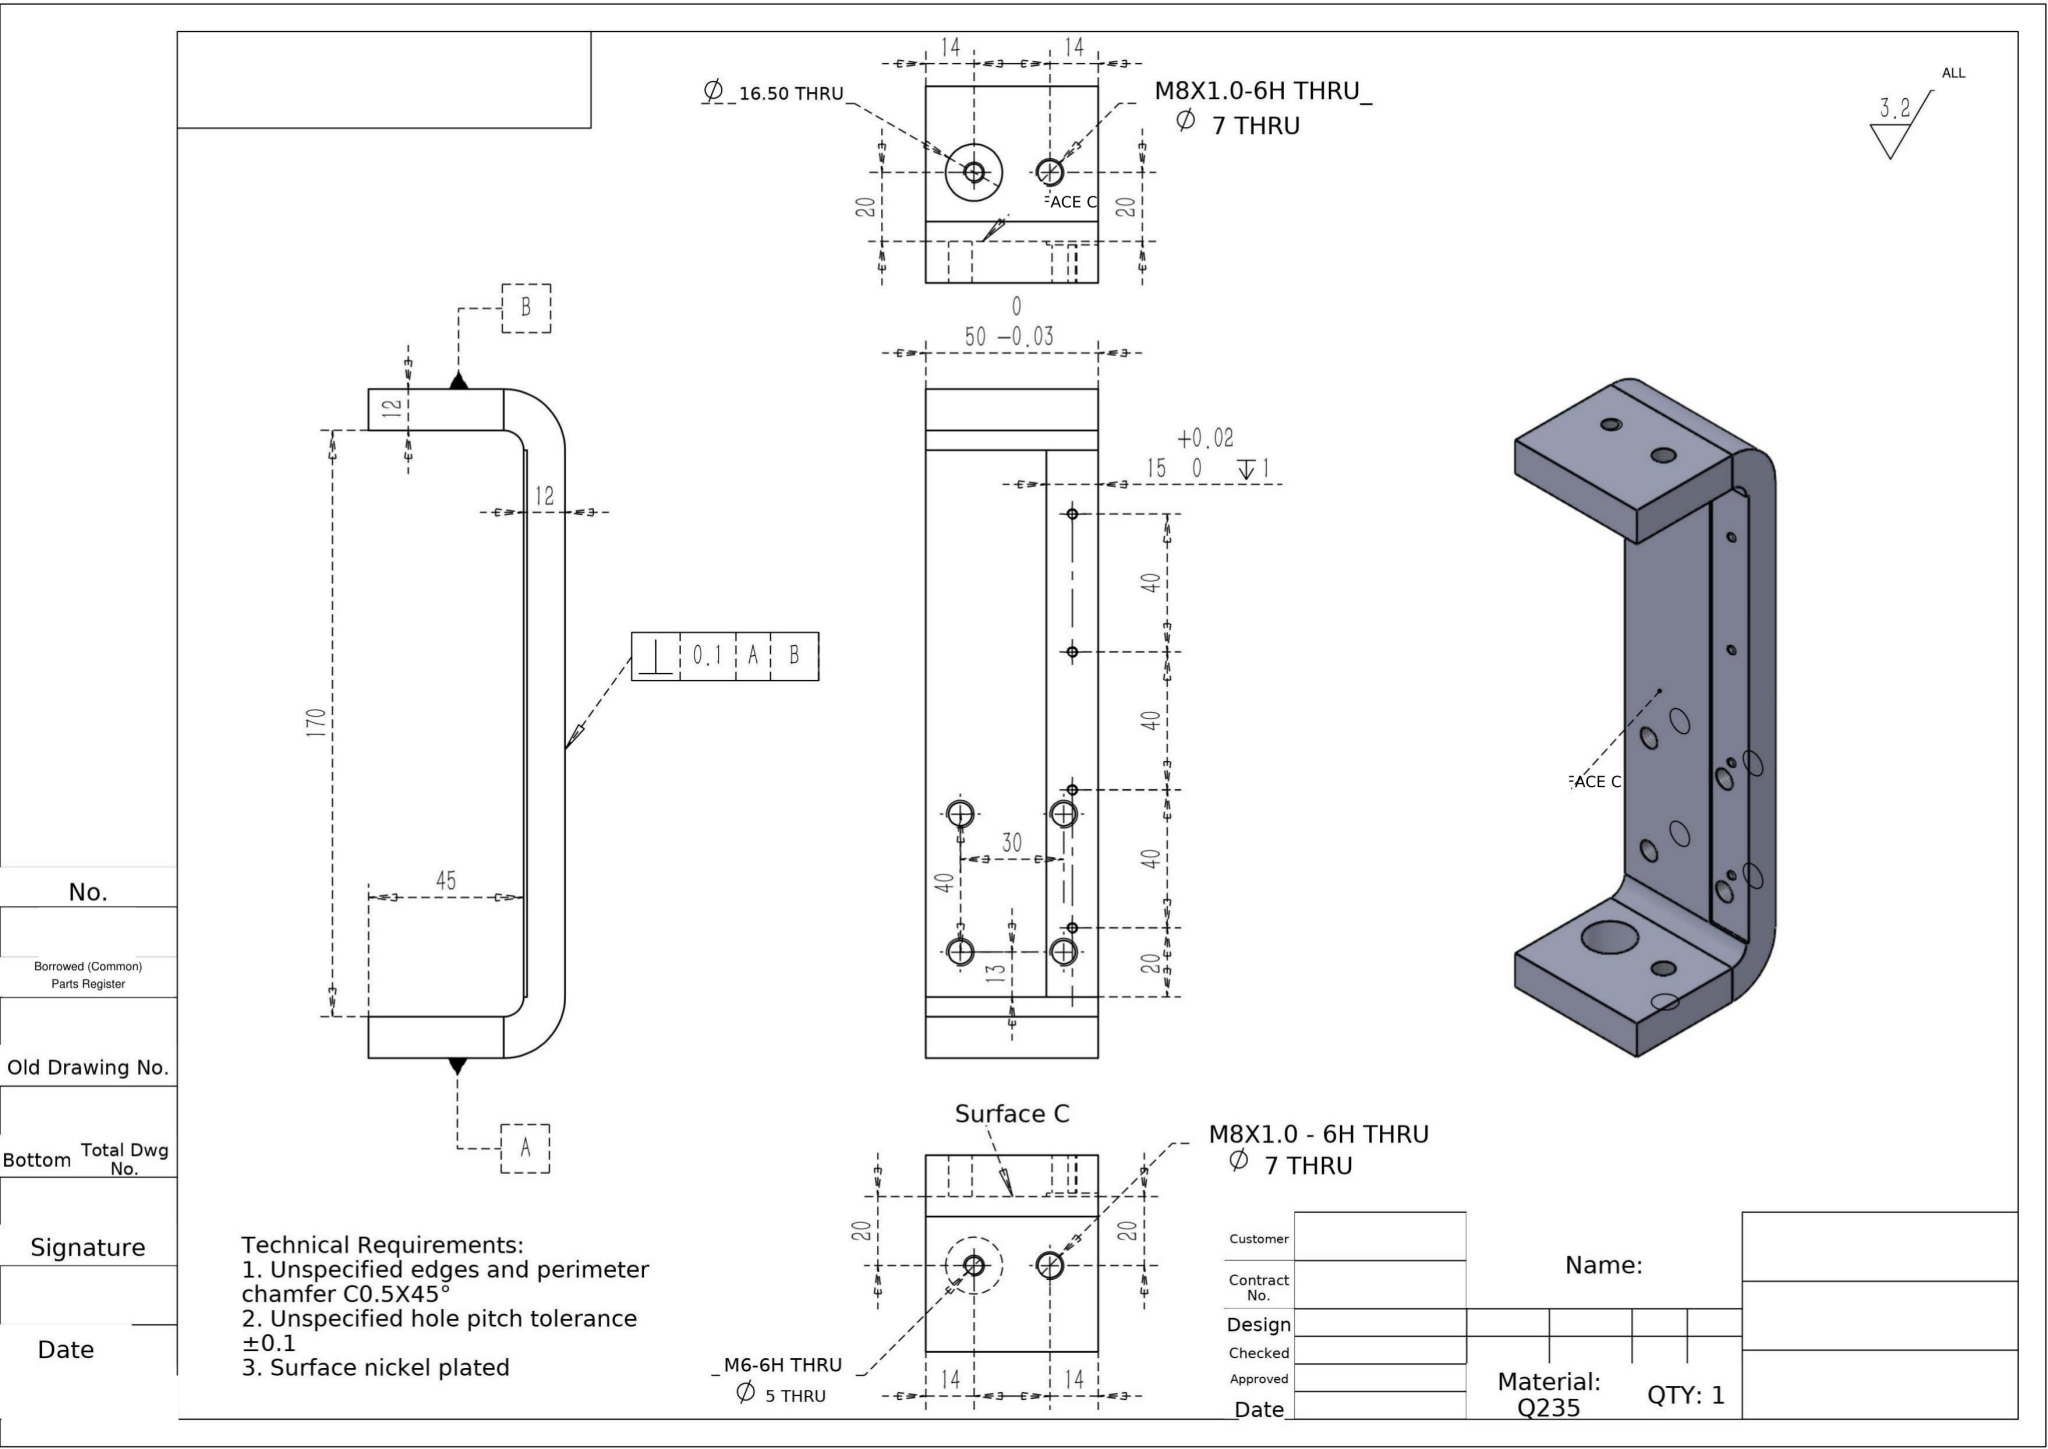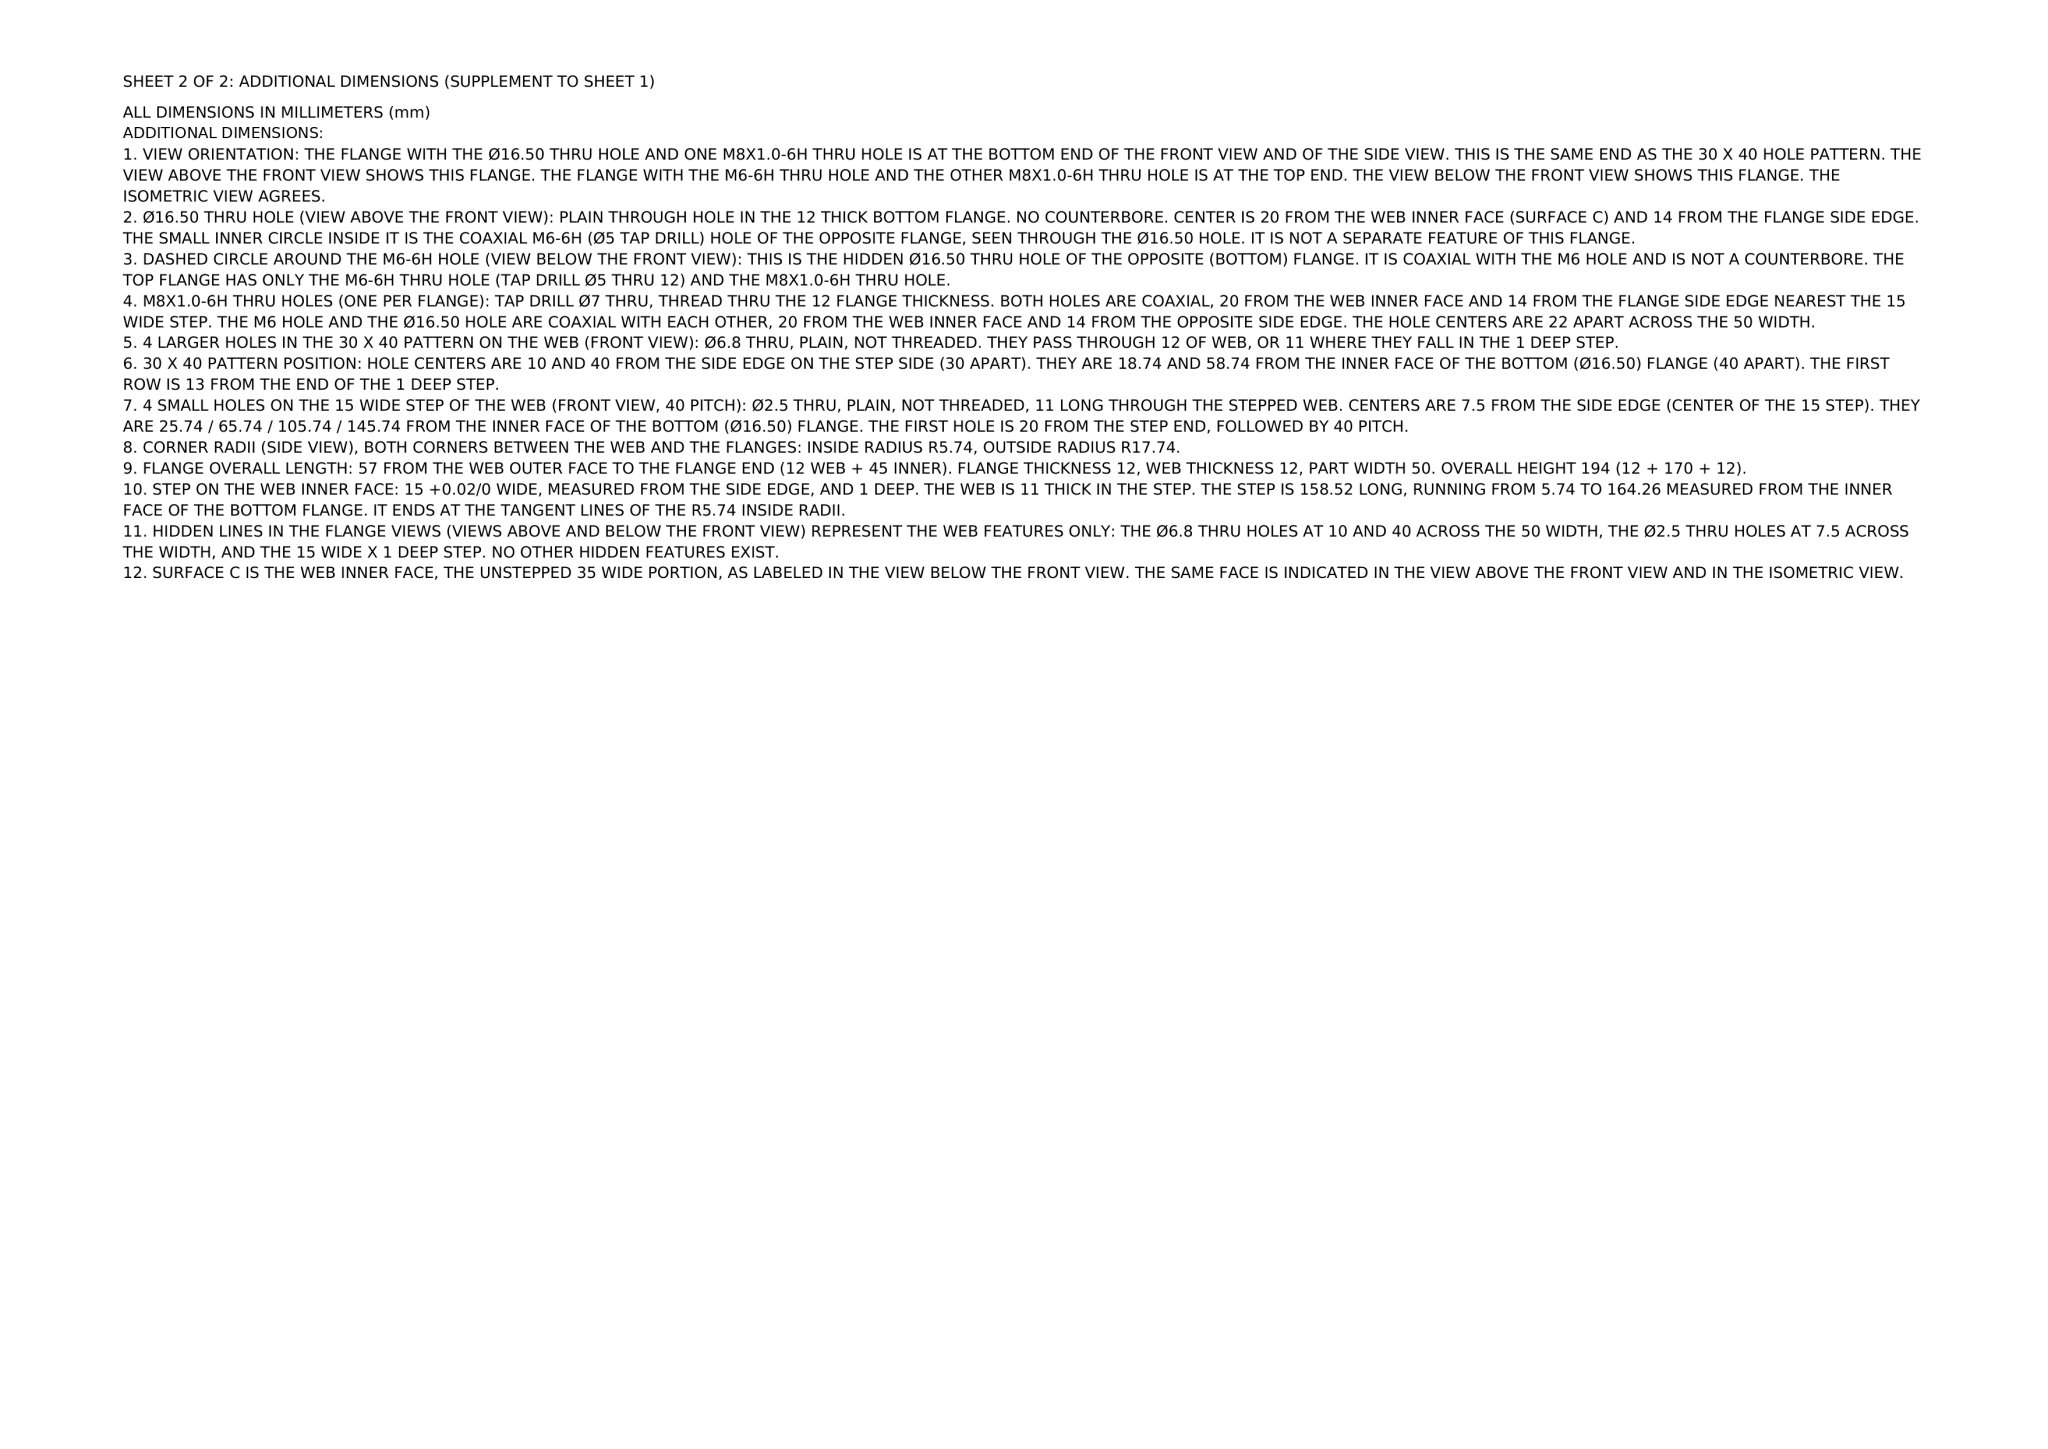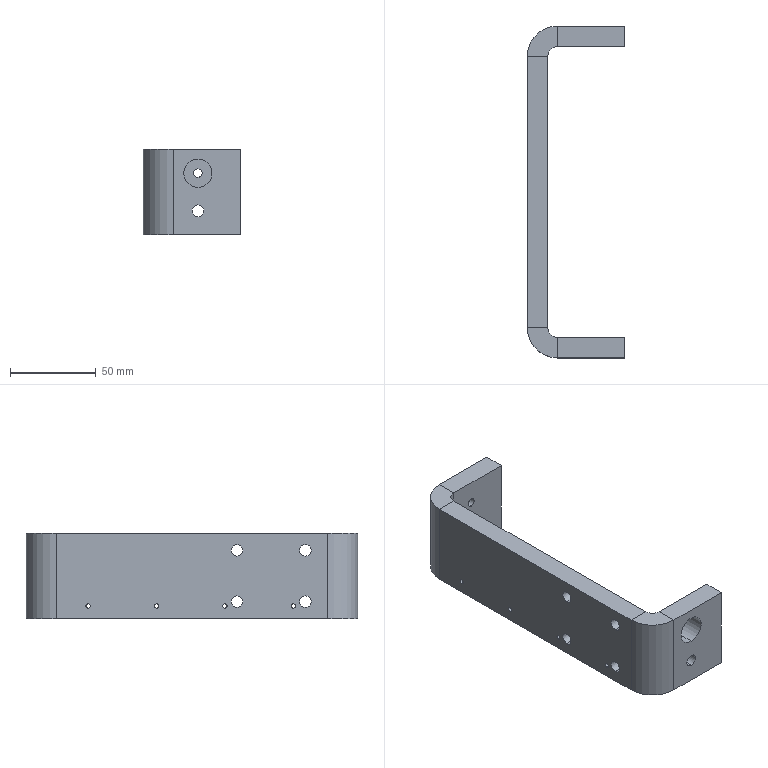Part | NX | mm | 1 solid | 48 faces | box 57 x 194 x 50 mm | volume 156366 mm3 | cylinder 28 | plane 20 | commonest cylinder face diameters 6.8 x8 2.5 x8 7 x4 16.5 x2 5 x2 11.473 x2 35.473 x2